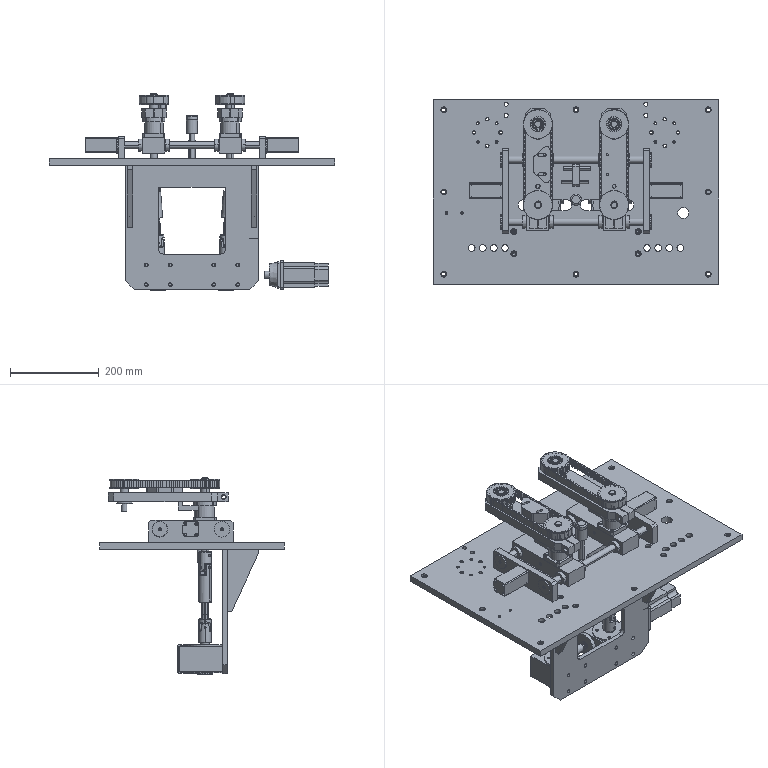Assembly | SolidWorks | mm | 71 component files | 71 solids | 3694 faces | box 643 x 415 x 442.5 mm | volume 8256780 mm3 | cylinder 1463 | plane 1317 | torus 376 | cone 330 | sphere 192 | spline 16 | commonest cylinder face diameters 5 x108 15 x106 6.5 x94 56 x84 62 x80 4 x68 9 x50 35 x50
Bill of materials:
400WMotor | 1 |  | Long prismatic body with a square cross-section and concave coved corners. One end has a square mounting flange with rounded corners and four corner through-holes. A short cylindrical shaft sticks out from a small round boss on the flange face. Its outline looks like a motor envelope, but that is a resemblance only.
AdjustmentNut | 1 |  | Plain hollow cylinder (tube or sleeve) with a concentric through-bore. It is somewhat taller than it is wide.
AdjustmentRod | 1 |  | Slender solid cylindrical rod or pin with small chamfers at both ends.
AxisEndCap | 6 |  | Thin flat disc with a small concentric central hole, like a washer. One outer edge appears chamfered.
BearingLM16LUU | 4 |  | Thick-walled cylindrical sleeve with a through-bore and two shallow external circumferential grooves, one near each end.
Connector | 1 |  | Square flange plate with chamfered corners, four corner holes and a large central circular opening. A cylindrical collar on one side tapers slightly and has an irregular, curved cut-out at its rim.
CrossJoint | 4 |  | Short cylindrical block with rounded/filleted end edges, an axial through-hole, and one machined flat on the side. A radial cross-hole runs through the flat.
DeepGrooveBallBearing6003_DeepGrooveBallBearing6003 | 4 |  | Ball-bearing-like ring assembly: concentric outer and inner rings with a single row of exposed balls between them and no visible shields or cage.
DeepGrooveBallBearing6202_DeepGrooveBallBearing6202 | 2 |  | Ball-bearing-like ring assembly: outer and inner rings with a single row of exposed balls and no visible shields. Compared with unnamed part it is somewhat wider relative to its diameter and has fewer balls.
DrivenWheel | 2 |  | Toothed pulley: a cylindrical hub with straight external teeth running parallel to the axis between two thin side flanges, and a plain central bore with an internal step or counterbore.
DriveWheel | 2 |  | Toothed pulley with two side flanges, similar to unnamed part, but with a smaller central bore that has a single keyway slot.
DriveWheelDriveShaft | 2 |  | Slender stepped shaft: a long main section, a larger-diameter collar near one end, and reduced-diameter end journals. Both ends have elongated slot or flat features, and there is a faint circumferential line near mid-length.
FilmPullingFixingSeat | 1 |  | Flat rectangular plate with a large rectangular window, two chamfered corners along one edge, and many small through holes.
FilmPullingFixingSeatSupportPlate | 2 |  | Tapered, wedge-shaped plate (gusset-like profile) with two holes in its wide end face.
FlangeClamp | 2 |  | L-shaped block: a flat base with a raised step at one end, one vertical through hole in the base, and a concave curved cutout at the other end.
GearboxShaft | 2 |  | Cylindrical pin with a thin round collar, a short larger-diameter end above the collar, and flat recesses along the shank.
GuidePlate | 2 |  | Rectangular block with one large vertical bore and four small holes around it, two large cross bores through the long side, and one small cross hole between them.
GuideRod | 2 |  | Long, slender cylindrical rod or tube with a small hole in the center of its end face.
LimitAdjustmentScrewRod | 2 |  | Plain solid cylindrical rod with flat ends.
PositioningScrewPlate | 1 |  | Thick rectangular block with two chamfered top corners and two through holes near the top edge.
RubberPad | 1 |  | Short stepped cylinder: a larger round head with a rounded top edge on a smaller cylindrical body, like a knob or cap.
SDA20X55 | 2 |  | Rectangular block with chamfered long edges, four holes in one end face, and a small stepped round boss sticking out of the other end.
ShaftSleeve | 2 |  | Hollow cylindrical tube with a square mounting flange that has four holes, plus a second round collar with small notches.
Spline | 2 |  | Shaft with lengthwise spline-like ribs, a shorter reduced-diameter end with a cross hole, and a small hole in the center of the end face.
SupportPlate | 2 |  | Rectangular flat bar/plate with two chamfered corners on one long edge, two larger through holes near the ends and a central pattern of one large hole surrounded by four smaller holes.
SynchronousBelt | 2 |  | Closed-loop oval (stadium-shaped) band with evenly spaced rectangular teeth along its inner face. The geometry looks like a toothed timing belt.
SynchronousBeltPressingBlock | 1 |  | Prismatic block with a tapered, roughly trapezoidal outline, rounded lobes at the corners, two parallel obround through slots and a small step along the flat back face.
TensionConnectionShaft | 2 |  | Stepped cylindrical pin/shaft with a larger-diameter central section, a smaller upper journal with a small groove near its end, a narrower neck and a lower shank. A transverse through hole and a flat-sided region are on the larger section.
TensionConnectionShaftPad | 1 |  | Flat circular ring (washer-like disc) with a central through hole and a chamfer on one outer edge.
UniversalJointA | 4 |  | Cylindrical sleeve with an axial through bore. One end is cut into two rounded tabs separated by a slot, each with a transverse hole, and a separate radial hole is in the full-diameter section.
UniversalJointB | 2 |  | Ring-shaped hub with a keyed bore (rectangular keyway notch). Two parallel legs extend from one face to form a U-shaped fork, with transverse holes in the legs and the hub wall.
UniversalJointC | 2 |  | Cylindrical shaft-like body ending in a two-pronged fork (clevis-like), with a cross hole in each prong. An internal toothed (spline-like) bore is visible at the base of the fork.
VerticalSealPanel | 1 |  | Large thin rectangular flat plate with many through holes: corner and edge holes, two circular bolt-circle patterns, rows of larger holes, one larger single hole and two collinear obround slots near the center.
WheelTensionAdjustmentPlate | 2 |  | Elongated flat arm with a split clamp at one end: a large bore with a slit running out to the end, and a transverse hole across the slit. The other end has chamfered corners, a long obround slot and three small holes in between.
WormGearReducerNRV30-10-L+R | 1 |  | Multi-body item: two similar box-shaped housings connected by a short shaft with a cylindrical sleeve or coupling. Each housing has a raised circular flange with four holes and a keyed central bore on one face, a round flange with a protruding shaft stub on a side face, and holes on its side faces.
Mates: